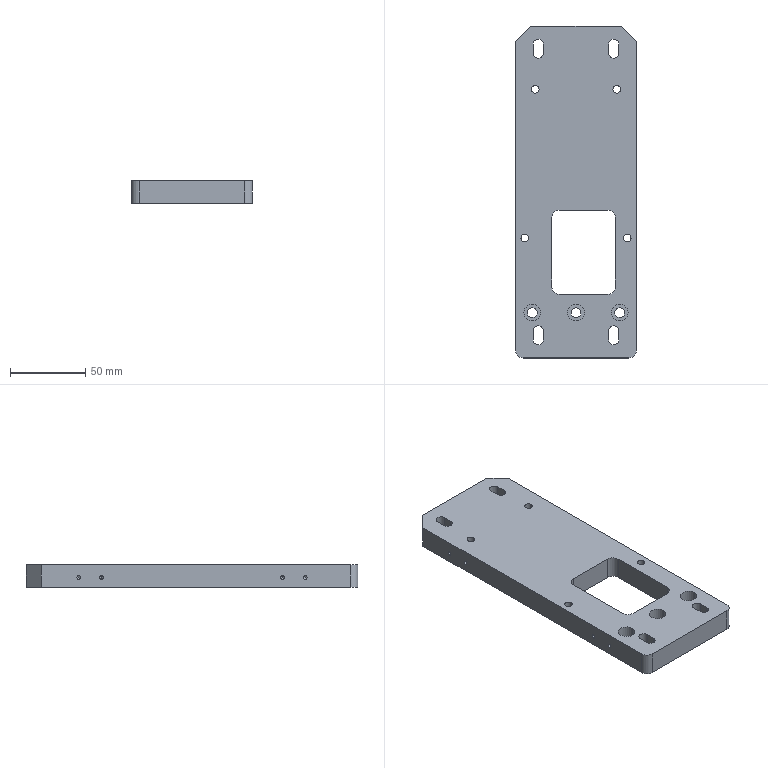CAM job | Mastercam | mm | 18 operations | part box 80 x 220 x 15
1. Facing | 20 - 63 平铣刀
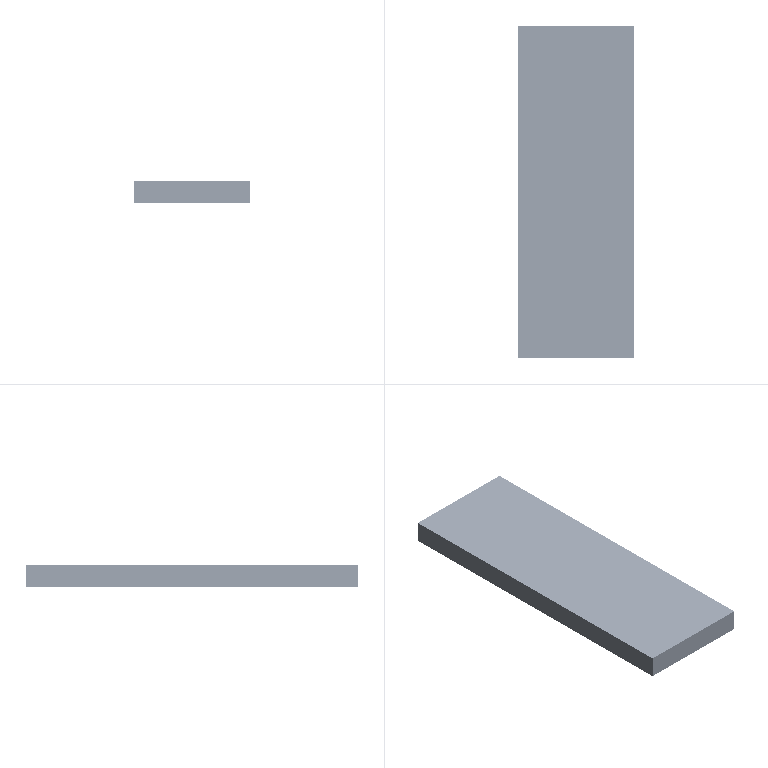2. Contour (Ramp) | 9 - 10 平铣刀
3. Contour (Ramp) | 9 - 10 平铣刀
4. 2D High Speed (2D Dynamic Mill) | 9 - 10 平铣刀
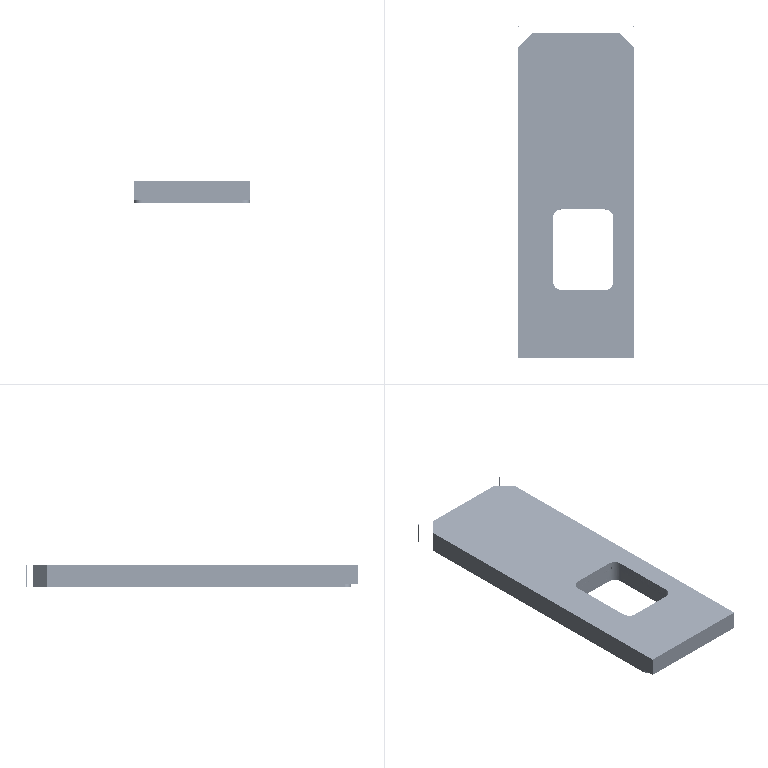5. Contour (2D) | 10 - 10 平铣刀
6. Contour (2D) | 10 - 10 平铣刀
7. Contour (Ramp) | 6 - 6 平铣刀
8. Contour (Ramp) | 6 - 6 平铣刀
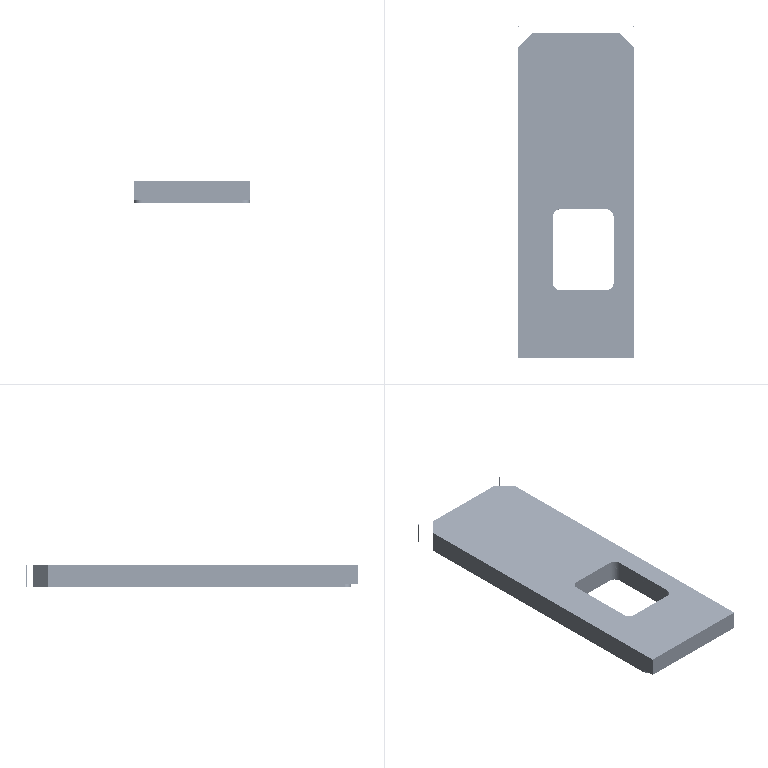9. Contour (Ramp) | 4 - 4 平铣刀
10. Contour (Ramp) | 4 - 4 平铣刀
11. Drill/Counterbore | 7 - 4 倒角刀
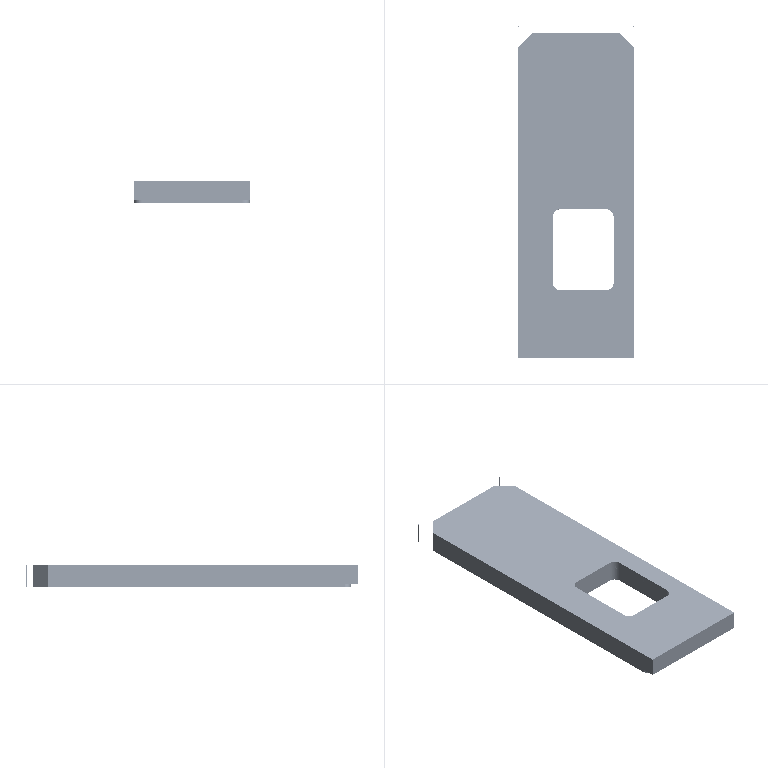12. Contour (2D chamfer) | 7 - 4 倒角刀
13. Facing | 20 - 63 平铣刀
14. Contour (Ramp) | 9 - 10 平铣刀
15. Contour (2D) | 10 - 10 平铣刀
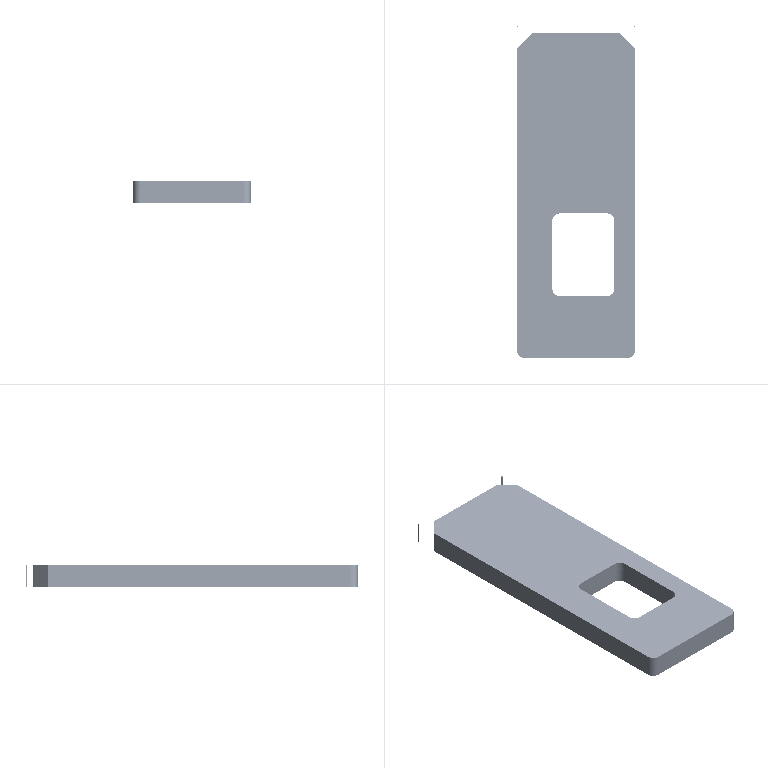16. Helix Bore | 6 - 6 平铣刀
17. Contour (2D chamfer) | 7 - 4 倒角刀
18. Drill/Counterbore | 7 - 4 倒角刀